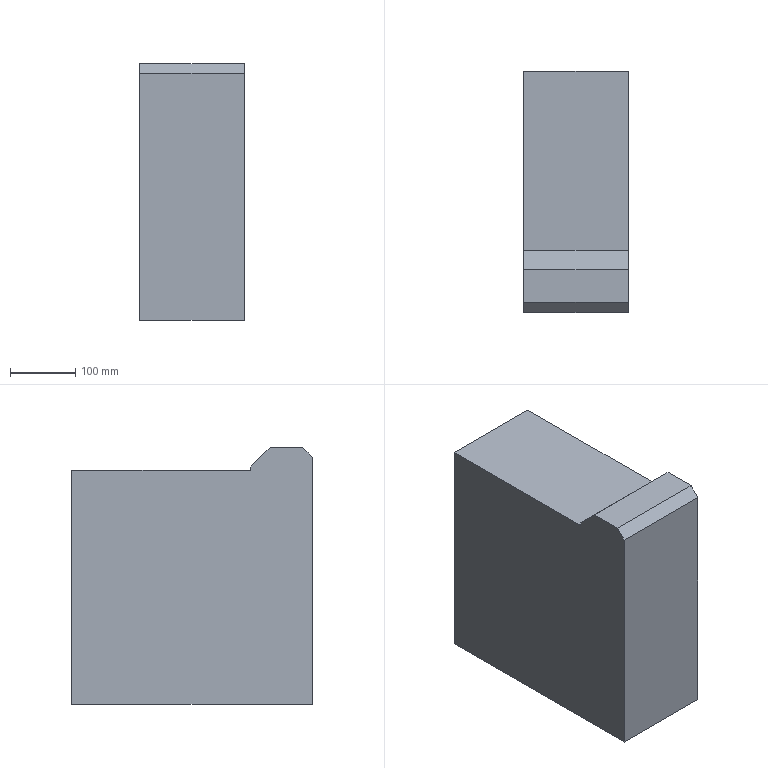Component | SolidWorks | Host-1 | 1 solid | 10 faces | box 160 x 370 x 395 mm | volume 21754000 mm3 | plane 10 | material Domestic 6061
build123d program:
from build123d import *

# Parameters (mm, degrees)
SKETCH1_W           = 160
SKETCH1_H           = 370
BOSS_EXTRUDE1_DEPTH = 360
SKETCH2_W           = 160
SKETCH2_H           = 95
BOSS_EXTRUDE2_DEPTH = 35
CHAMFER1_SIZE       = 15
CHAMFER2_SIZE       = 30


with BuildPart() as part:
    # Sketch1 → Boss-Extrude1 (new body)
    with BuildSketch(Plane.XY):
        Rectangle(SKETCH1_W, SKETCH1_H)
    extrude(amount=BOSS_EXTRUDE1_DEPTH)

    # Sketch2 → Boss-Extrude2 (add)
    with BuildSketch(Plane.XY.offset(360)):
        with Locations((0, -137.5)):
            Rectangle(SKETCH2_W, SKETCH2_H)
    extrude(amount=BOSS_EXTRUDE2_DEPTH)

    # Chamfer1
    chamfer1_edges = [part.edges().sort_by_distance(p)[0] for p in [
        (0, -185, 395),
    ]]
    chamfer(chamfer1_edges, length=CHAMFER1_SIZE)

    # Chamfer2
    chamfer2_edges = [part.edges().sort_by_distance(p)[0] for p in [
        (0, -90, 395),
    ]]
    chamfer(chamfer2_edges, length=CHAMFER2_SIZE)


solid = part.part

# Placed as in the assembly
solid = solid.moved(Location((-204.631, 220, 55), (0, 0, 0)))
STEP:
#1=COLOUR_RGB('',0.7922,0.8196,0.9333);
#2=FILL_AREA_STYLE_COLOUR('',#1);
#3=FILL_AREA_STYLE('',(#2));
#4=SURFACE_STYLE_FILL_AREA(#3);
#5=SURFACE_SIDE_STYLE('',(#4));
#6=SURFACE_STYLE_USAGE(.BOTH.,#5);
#7=PRESENTATION_STYLE_ASSIGNMENT((#6));
#8=CARTESIAN_POINT('',(-4.907,5.118,16.535));
#9=VERTEX_POINT('',#8);
#10=CARTESIAN_POINT('',(-4.907,5.118,16.339));
#11=VERTEX_POINT('',#10);
#12=CARTESIAN_POINT('',(-4.907,5.118,17.717));
#13=DIRECTION('',(0.,0.,-1.));
#14=VECTOR('',#13,39.37);
#15=LINE('',#12,#14);
#16=EDGE_CURVE('',#9,#11,#15,.T.);
#17=ORIENTED_EDGE('',*,*,#16,.F.);
#18=CARTESIAN_POINT('',(-4.907,3.937,17.717));
#19=VERTEX_POINT('',#18);
#20=CARTESIAN_POINT('',(-4.907,3.937,17.717));
#21=DIRECTION('',(0.,-0.7071,0.7071));
#22=VECTOR('',#21,39.37);
#23=LINE('',#20,#22);
#24=EDGE_CURVE('',#9,#19,#23,.T.);
#25=ORIENTED_EDGE('',*,*,#24,.T.);
#26=CARTESIAN_POINT('',(-4.907,1.969,17.717));
#27=VERTEX_POINT('',#26);
#28=CARTESIAN_POINT('',(-4.907,5.118,17.717));
#29=DIRECTION('',(-0.,1.,0.));
#30=VECTOR('',#29,39.37);
#31=LINE('',#28,#30);
#32=EDGE_CURVE('',#27,#19,#31,.T.);
#33=ORIENTED_EDGE('',*,*,#32,.F.);
#34=CARTESIAN_POINT('',(-4.907,1.378,17.126));
#35=VERTEX_POINT('',#34);
#36=CARTESIAN_POINT('',(-4.907,1.969,17.717));
#37=DIRECTION('',(0.,-0.7071,-0.7071));
#38=VECTOR('',#37,39.37);
#39=LINE('',#36,#38);
#40=EDGE_CURVE('',#27,#35,#39,.T.);
#41=ORIENTED_EDGE('',*,*,#40,.T.);
#42=CARTESIAN_POINT('',(-4.907,1.378,2.165));
#43=VERTEX_POINT('',#42);
#44=CARTESIAN_POINT('',(-4.907,1.378,16.339));
#45=DIRECTION('',(0.,0.,-1.));
#46=VECTOR('',#45,39.37);
#47=LINE('',#44,#46);
#48=EDGE_CURVE('',#35,#43,#47,.T.);
#49=ORIENTED_EDGE('',*,*,#48,.T.);
#50=CARTESIAN_POINT('',(-4.907,15.945,2.165));
#51=VERTEX_POINT('',#50);
#52=CARTESIAN_POINT('',(-4.907,15.945,2.165));
#53=DIRECTION('',(-0.,1.,0.));
#54=VECTOR('',#53,39.37);
#55=LINE('',#52,#54);
#56=EDGE_CURVE('',#43,#51,#55,.T.);
#57=ORIENTED_EDGE('',*,*,#56,.T.);
#58=CARTESIAN_POINT('',(-4.907,15.945,16.339));
#59=VERTEX_POINT('',#58);
#60=CARTESIAN_POINT('',(-4.907,15.945,16.339));
#61=DIRECTION('',(0.,0.,-1.));
#62=VECTOR('',#61,39.37);
#63=LINE('',#60,#62);
#64=EDGE_CURVE('',#59,#51,#63,.T.);
#65=ORIENTED_EDGE('',*,*,#64,.F.);
#66=CARTESIAN_POINT('',(-4.907,15.945,16.339));
#67=DIRECTION('',(-0.,1.,0.));
#68=VECTOR('',#67,39.37);
#69=LINE('',#66,#68);
#70=EDGE_CURVE('',#11,#59,#69,.T.);
#71=ORIENTED_EDGE('',*,*,#70,.F.);
#72=EDGE_LOOP('',(#17,#25,#33,#41,#49,#57,#65,#71));
#73=FACE_OUTER_BOUND('',#72,.T.);
#74=CARTESIAN_POINT('',(-4.907,15.945,16.339));
#75=DIRECTION('',(-1.,-0.,0.));
#76=DIRECTION('',(0.,-1.,0.));
#77=AXIS2_PLACEMENT_3D('',#74,#75,#76);
#78=PLANE('',#77);
#79=ADVANCED_FACE('',(#73),#78,.F.);
#80=CARTESIAN_POINT('',(-11.206,15.945,2.165));
#81=VERTEX_POINT('',#80);
#82=CARTESIAN_POINT('',(-11.206,15.945,2.165));
#83=DIRECTION('',(-1.,0.,0.));
#84=VECTOR('',#83,39.37);
#85=LINE('',#82,#84);
#86=EDGE_CURVE('',#51,#81,#85,.T.);
#87=ORIENTED_EDGE('',*,*,#86,.T.);
#88=CARTESIAN_POINT('',(-11.206,15.945,16.339));
#89=VERTEX_POINT('',#88);
#90=CARTESIAN_POINT('',(-11.206,15.945,16.339));
#91=DIRECTION('',(0.,0.,-1.));
#92=VECTOR('',#91,39.37);
#93=LINE('',#90,#92);
#94=EDGE_CURVE('',#89,#81,#93,.T.);
#95=ORIENTED_EDGE('',*,*,#94,.F.);
#96=CARTESIAN_POINT('',(-11.206,15.945,16.339));
#97=DIRECTION('',(-1.,0.,0.));
#98=VECTOR('',#97,39.37);
#99=LINE('',#96,#98);
#100=EDGE_CURVE('',#59,#89,#99,.T.);
#101=ORIENTED_EDGE('',*,*,#100,.F.);
#102=ORIENTED_EDGE('',*,*,#64,.T.);
#103=EDGE_LOOP('',(#87,#95,#101,#102));
#104=FACE_OUTER_BOUND('',#103,.T.);
#105=CARTESIAN_POINT('',(-11.206,15.945,16.339));
#106=DIRECTION('',(0.,-1.,0.));
#107=DIRECTION('',(0.,0.,-1.));
#108=AXIS2_PLACEMENT_3D('',#105,#106,#107);
#109=PLANE('',#108);
#110=ADVANCED_FACE('',(#104),#109,.F.);
#111=CARTESIAN_POINT('',(-11.206,3.937,17.717));
#112=VERTEX_POINT('',#111);
#113=CARTESIAN_POINT('',(-11.206,1.969,17.717));
#114=VERTEX_POINT('',#113);
#115=CARTESIAN_POINT('',(-11.206,5.118,17.717));
#116=DIRECTION('',(0.,-1.,0.));
#117=VECTOR('',#116,39.37);
#118=LINE('',#115,#117);
#119=EDGE_CURVE('',#112,#114,#118,.T.);
#120=ORIENTED_EDGE('',*,*,#119,.F.);
#121=CARTESIAN_POINT('',(-11.206,5.118,16.535));
#122=VERTEX_POINT('',#121);
#123=CARTESIAN_POINT('',(-11.206,3.937,17.717));
#124=DIRECTION('',(-0.,0.7071,-0.7071));
#125=VECTOR('',#124,39.37);
#126=LINE('',#123,#125);
#127=EDGE_CURVE('',#112,#122,#126,.T.);
#128=ORIENTED_EDGE('',*,*,#127,.T.);
#129=CARTESIAN_POINT('',(-11.206,5.118,16.339));
#130=VERTEX_POINT('',#129);
#131=CARTESIAN_POINT('',(-11.206,5.118,17.717));
#132=DIRECTION('',(0.,0.,-1.));
#133=VECTOR('',#132,39.37);
#134=LINE('',#131,#133);
#135=EDGE_CURVE('',#122,#130,#134,.T.);
#136=ORIENTED_EDGE('',*,*,#135,.T.);
#137=CARTESIAN_POINT('',(-11.206,15.945,16.339));
#138=DIRECTION('',(0.,-1.,0.));
#139=VECTOR('',#138,39.37);
#140=LINE('',#137,#139);
#141=EDGE_CURVE('',#89,#130,#140,.T.);
#142=ORIENTED_EDGE('',*,*,#141,.F.);
#143=ORIENTED_EDGE('',*,*,#94,.T.);
#144=CARTESIAN_POINT('',(-11.206,1.378,2.165));
#145=VERTEX_POINT('',#144);
#146=CARTESIAN_POINT('',(-11.206,15.945,2.165));
#147=DIRECTION('',(0.,-1.,0.));
#148=VECTOR('',#147,39.37);
#149=LINE('',#146,#148);
#150=EDGE_CURVE('',#81,#145,#149,.T.);
#151=ORIENTED_EDGE('',*,*,#150,.T.);
#152=CARTESIAN_POINT('',(-11.206,1.378,17.126));
#153=VERTEX_POINT('',#152);
#154=CARTESIAN_POINT('',(-11.206,1.378,16.339));
#155=DIRECTION('',(0.,0.,-1.));
#156=VECTOR('',#155,39.37);
#157=LINE('',#154,#156);
#158=EDGE_CURVE('',#153,#145,#157,.T.);
#159=ORIENTED_EDGE('',*,*,#158,.F.);
#160=CARTESIAN_POINT('',(-11.206,1.969,17.717));
#161=DIRECTION('',(-0.,0.7071,0.7071));
#162=VECTOR('',#161,39.37);
#163=LINE('',#160,#162);
#164=EDGE_CURVE('',#153,#114,#163,.T.);
#165=ORIENTED_EDGE('',*,*,#164,.T.);
#166=EDGE_LOOP('',(#120,#128,#136,#142,#143,#151,#159,#165));
#167=FACE_OUTER_BOUND('',#166,.T.);
#168=CARTESIAN_POINT('',(-11.206,15.945,16.339));
#169=DIRECTION('',(1.,0.,0.));
#170=DIRECTION('',(-0.,1.,0.));
#171=AXIS2_PLACEMENT_3D('',#168,#169,#170);
#172=PLANE('',#171);
#173=ADVANCED_FACE('',(#167),#172,.F.);
#174=ORIENTED_EDGE('',*,*,#48,.F.);
#175=CARTESIAN_POINT('',(-11.206,1.378,17.126));
#176=DIRECTION('',(-1.,0.,0.));
#177=VECTOR('',#176,39.37);
#178=LINE('',#175,#177);
#179=EDGE_CURVE('',#35,#153,#178,.T.);
#180=ORIENTED_EDGE('',*,*,#179,.T.);
#181=ORIENTED_EDGE('',*,*,#158,.T.);
#182=CARTESIAN_POINT('',(-11.206,1.378,2.165));
#183=DIRECTION('',(1.,0.,0.));
#184=VECTOR('',#183,39.37);
#185=LINE('',#182,#184);
#186=EDGE_CURVE('',#145,#43,#185,.T.);
#187=ORIENTED_EDGE('',*,*,#186,.T.);
#188=EDGE_LOOP('',(#174,#180,#181,#187));
#189=FACE_OUTER_BOUND('',#188,.T.);
#190=CARTESIAN_POINT('',(-11.206,1.378,16.339));
#191=DIRECTION('',(0.,1.,0.));
#192=DIRECTION('',(0.,0.,1.));
#193=AXIS2_PLACEMENT_3D('',#190,#191,#192);
#194=PLANE('',#193);
#195=ADVANCED_FACE('',(#189),#194,.F.);
#196=CARTESIAN_POINT('',(-11.206,5.118,16.339));
#197=DIRECTION('',(-1.,0.,0.));
#198=VECTOR('',#197,39.37);
#199=LINE('',#196,#198);
#200=EDGE_CURVE('',#11,#130,#199,.T.);
#201=ORIENTED_EDGE('',*,*,#200,.F.);
#202=ORIENTED_EDGE('',*,*,#70,.T.);
#203=ORIENTED_EDGE('',*,*,#100,.T.);
#204=ORIENTED_EDGE('',*,*,#141,.T.);
#205=EDGE_LOOP('',(#201,#202,#203,#204));
#206=FACE_OUTER_BOUND('',#205,.T.);
#207=CARTESIAN_POINT('',(-4.907,1.378,16.339));
#208=DIRECTION('',(0.,0.,1.));
#209=DIRECTION('',(1.,0.,0.));
#210=AXIS2_PLACEMENT_3D('',#207,#208,#209);
#211=PLANE('',#210);
#212=ADVANCED_FACE('',(#206),#211,.T.);
#213=ORIENTED_EDGE('',*,*,#56,.F.);
#214=ORIENTED_EDGE('',*,*,#186,.F.);
#215=ORIENTED_EDGE('',*,*,#150,.F.);
#216=ORIENTED_EDGE('',*,*,#86,.F.);
#217=EDGE_LOOP('',(#213,#214,#215,#216));
#218=FACE_OUTER_BOUND('',#217,.T.);
#219=CARTESIAN_POINT('',(-4.907,1.378,2.165));
#220=DIRECTION('',(0.,0.,1.));
#221=DIRECTION('',(1.,0.,0.));
#222=AXIS2_PLACEMENT_3D('',#219,#220,#221);
#223=PLANE('',#222);
#224=ADVANCED_FACE('',(#218),#223,.F.);
#225=ORIENTED_EDGE('',*,*,#135,.F.);
#226=CARTESIAN_POINT('',(-4.907,5.118,16.535));
#227=DIRECTION('',(1.,0.,0.));
#228=VECTOR('',#227,39.37);
#229=LINE('',#226,#228);
#230=EDGE_CURVE('',#122,#9,#229,.T.);
#231=ORIENTED_EDGE('',*,*,#230,.T.);
#232=ORIENTED_EDGE('',*,*,#16,.T.);
#233=ORIENTED_EDGE('',*,*,#200,.T.);
#234=EDGE_LOOP('',(#225,#231,#232,#233));
#235=FACE_OUTER_BOUND('',#234,.T.);
#236=CARTESIAN_POINT('',(-11.206,5.118,17.717));
#237=DIRECTION('',(0.,-1.,0.));
#238=DIRECTION('',(0.,0.,-1.));
#239=AXIS2_PLACEMENT_3D('',#236,#237,#238);
#240=PLANE('',#239);
#241=ADVANCED_FACE('',(#235),#240,.F.);
#242=ORIENTED_EDGE('',*,*,#32,.T.);
#243=CARTESIAN_POINT('',(-11.206,3.937,17.717));
#244=DIRECTION('',(-1.,0.,0.));
#245=VECTOR('',#244,39.37);
#246=LINE('',#243,#245);
#247=EDGE_CURVE('',#19,#112,#246,.T.);
#248=ORIENTED_EDGE('',*,*,#247,.T.);
#249=ORIENTED_EDGE('',*,*,#119,.T.);
#250=CARTESIAN_POINT('',(-4.907,1.969,17.717));
#251=DIRECTION('',(1.,0.,0.));
#252=VECTOR('',#251,39.37);
#253=LINE('',#250,#252);
#254=EDGE_CURVE('',#114,#27,#253,.T.);
#255=ORIENTED_EDGE('',*,*,#254,.T.);
#256=EDGE_LOOP('',(#242,#248,#249,#255));
#257=FACE_OUTER_BOUND('',#256,.T.);
#258=CARTESIAN_POINT('',(-4.907,1.378,17.717));
#259=DIRECTION('',(0.,0.,1.));
#260=DIRECTION('',(1.,0.,0.));
#261=AXIS2_PLACEMENT_3D('',#258,#259,#260);
#262=PLANE('',#261);
#263=ADVANCED_FACE('',(#257),#262,.T.);
#264=ORIENTED_EDGE('',*,*,#164,.F.);
#265=ORIENTED_EDGE('',*,*,#179,.F.);
#266=ORIENTED_EDGE('',*,*,#40,.F.);
#267=ORIENTED_EDGE('',*,*,#254,.F.);
#268=EDGE_LOOP('',(#264,#265,#266,#267));
#269=FACE_OUTER_BOUND('',#268,.T.);
#270=CARTESIAN_POINT('',(-4.907,1.969,17.717));
#271=DIRECTION('',(0.,-0.7071,0.7071));
#272=DIRECTION('',(0.,-0.7071,-0.7071));
#273=AXIS2_PLACEMENT_3D('',#270,#271,#272);
#274=PLANE('',#273);
#275=ADVANCED_FACE('',(#269),#274,.T.);
#276=ORIENTED_EDGE('',*,*,#24,.F.);
#277=ORIENTED_EDGE('',*,*,#230,.F.);
#278=ORIENTED_EDGE('',*,*,#127,.F.);
#279=ORIENTED_EDGE('',*,*,#247,.F.);
#280=EDGE_LOOP('',(#276,#277,#278,#279));
#281=FACE_OUTER_BOUND('',#280,.T.);
#282=CARTESIAN_POINT('',(-4.907,3.937,17.717));
#283=DIRECTION('',(0.,0.7071,0.7071));
#284=DIRECTION('',(0.,-0.7071,0.7071));
#285=AXIS2_PLACEMENT_3D('',#282,#283,#284);
#286=PLANE('',#285);
#287=ADVANCED_FACE('',(#281),#286,.T.);
#288=CLOSED_SHELL('',(#79,#110,#173,#195,#212,#224,#241,#263,#275,#287));
#289=MANIFOLD_SOLID_BREP('',#288);
#290=STYLED_ITEM('',(#7),#289);
#291=PRESENTATION_LAYER_ASSIGNMENT('','',(#290));
#292=(LENGTH_UNIT()NAMED_UNIT(*)SI_UNIT($,.METRE.));
#293=LENGTH_MEASURE_WITH_UNIT(LENGTH_MEASURE(0.0254),#292);
#294=DIMENSIONAL_EXPONENTS(1.,0.,0.,0.,0.,0.,0.);
#295=(CONVERSION_BASED_UNIT('',#293)LENGTH_UNIT()NAMED_UNIT(#294));
#296=UNCERTAINTY_MEASURE_WITH_UNIT(LENGTH_MEASURE(0.00001),#295,'','');
#297=(NAMED_UNIT(*)PLANE_ANGLE_UNIT()SI_UNIT($,.RADIAN.));
#298=(NAMED_UNIT(*)SI_UNIT($,.STERADIAN.)SOLID_ANGLE_UNIT());
#299=(GEOMETRIC_REPRESENTATION_CONTEXT(3)GLOBAL_UNCERTAINTY_ASSIGNED_CONTEXT((#296))GLOBAL_UNIT_ASSIGNED_CONTEXT((#295,#297,#298))REPRESENTATION_CONTEXT('',''));
#300=MECHANICAL_DESIGN_GEOMETRIC_PRESENTATION_REPRESENTATION('',(#290),#299);
#301=CARTESIAN_POINT('',(0.,0.,0.));
#302=DIRECTION('',(0.,0.,1.));
#303=DIRECTION('',(1.,0.,0.));
#304=AXIS2_PLACEMENT_3D('',#301,#302,#303);
#305=(LENGTH_UNIT()NAMED_UNIT(*)SI_UNIT($,.METRE.));
#306=LENGTH_MEASURE_WITH_UNIT(LENGTH_MEASURE(0.0254),#305);
#307=DIMENSIONAL_EXPONENTS(1.,0.,0.,0.,0.,0.,0.);
#308=(CONVERSION_BASED_UNIT('',#306)LENGTH_UNIT()NAMED_UNIT(#307));
#309=UNCERTAINTY_MEASURE_WITH_UNIT(LENGTH_MEASURE(0.00001),#308,'','');
#310=(NAMED_UNIT(*)PLANE_ANGLE_UNIT()SI_UNIT($,.RADIAN.));
#311=(NAMED_UNIT(*)SI_UNIT($,.STERADIAN.)SOLID_ANGLE_UNIT());
#312=(GEOMETRIC_REPRESENTATION_CONTEXT(3)GLOBAL_UNCERTAINTY_ASSIGNED_CONTEXT((#309))GLOBAL_UNIT_ASSIGNED_CONTEXT((#308,#310,#311))REPRESENTATION_CONTEXT('',''));
#313=ADVANCED_BREP_SHAPE_REPRESENTATION('',(#289,#304),#312);